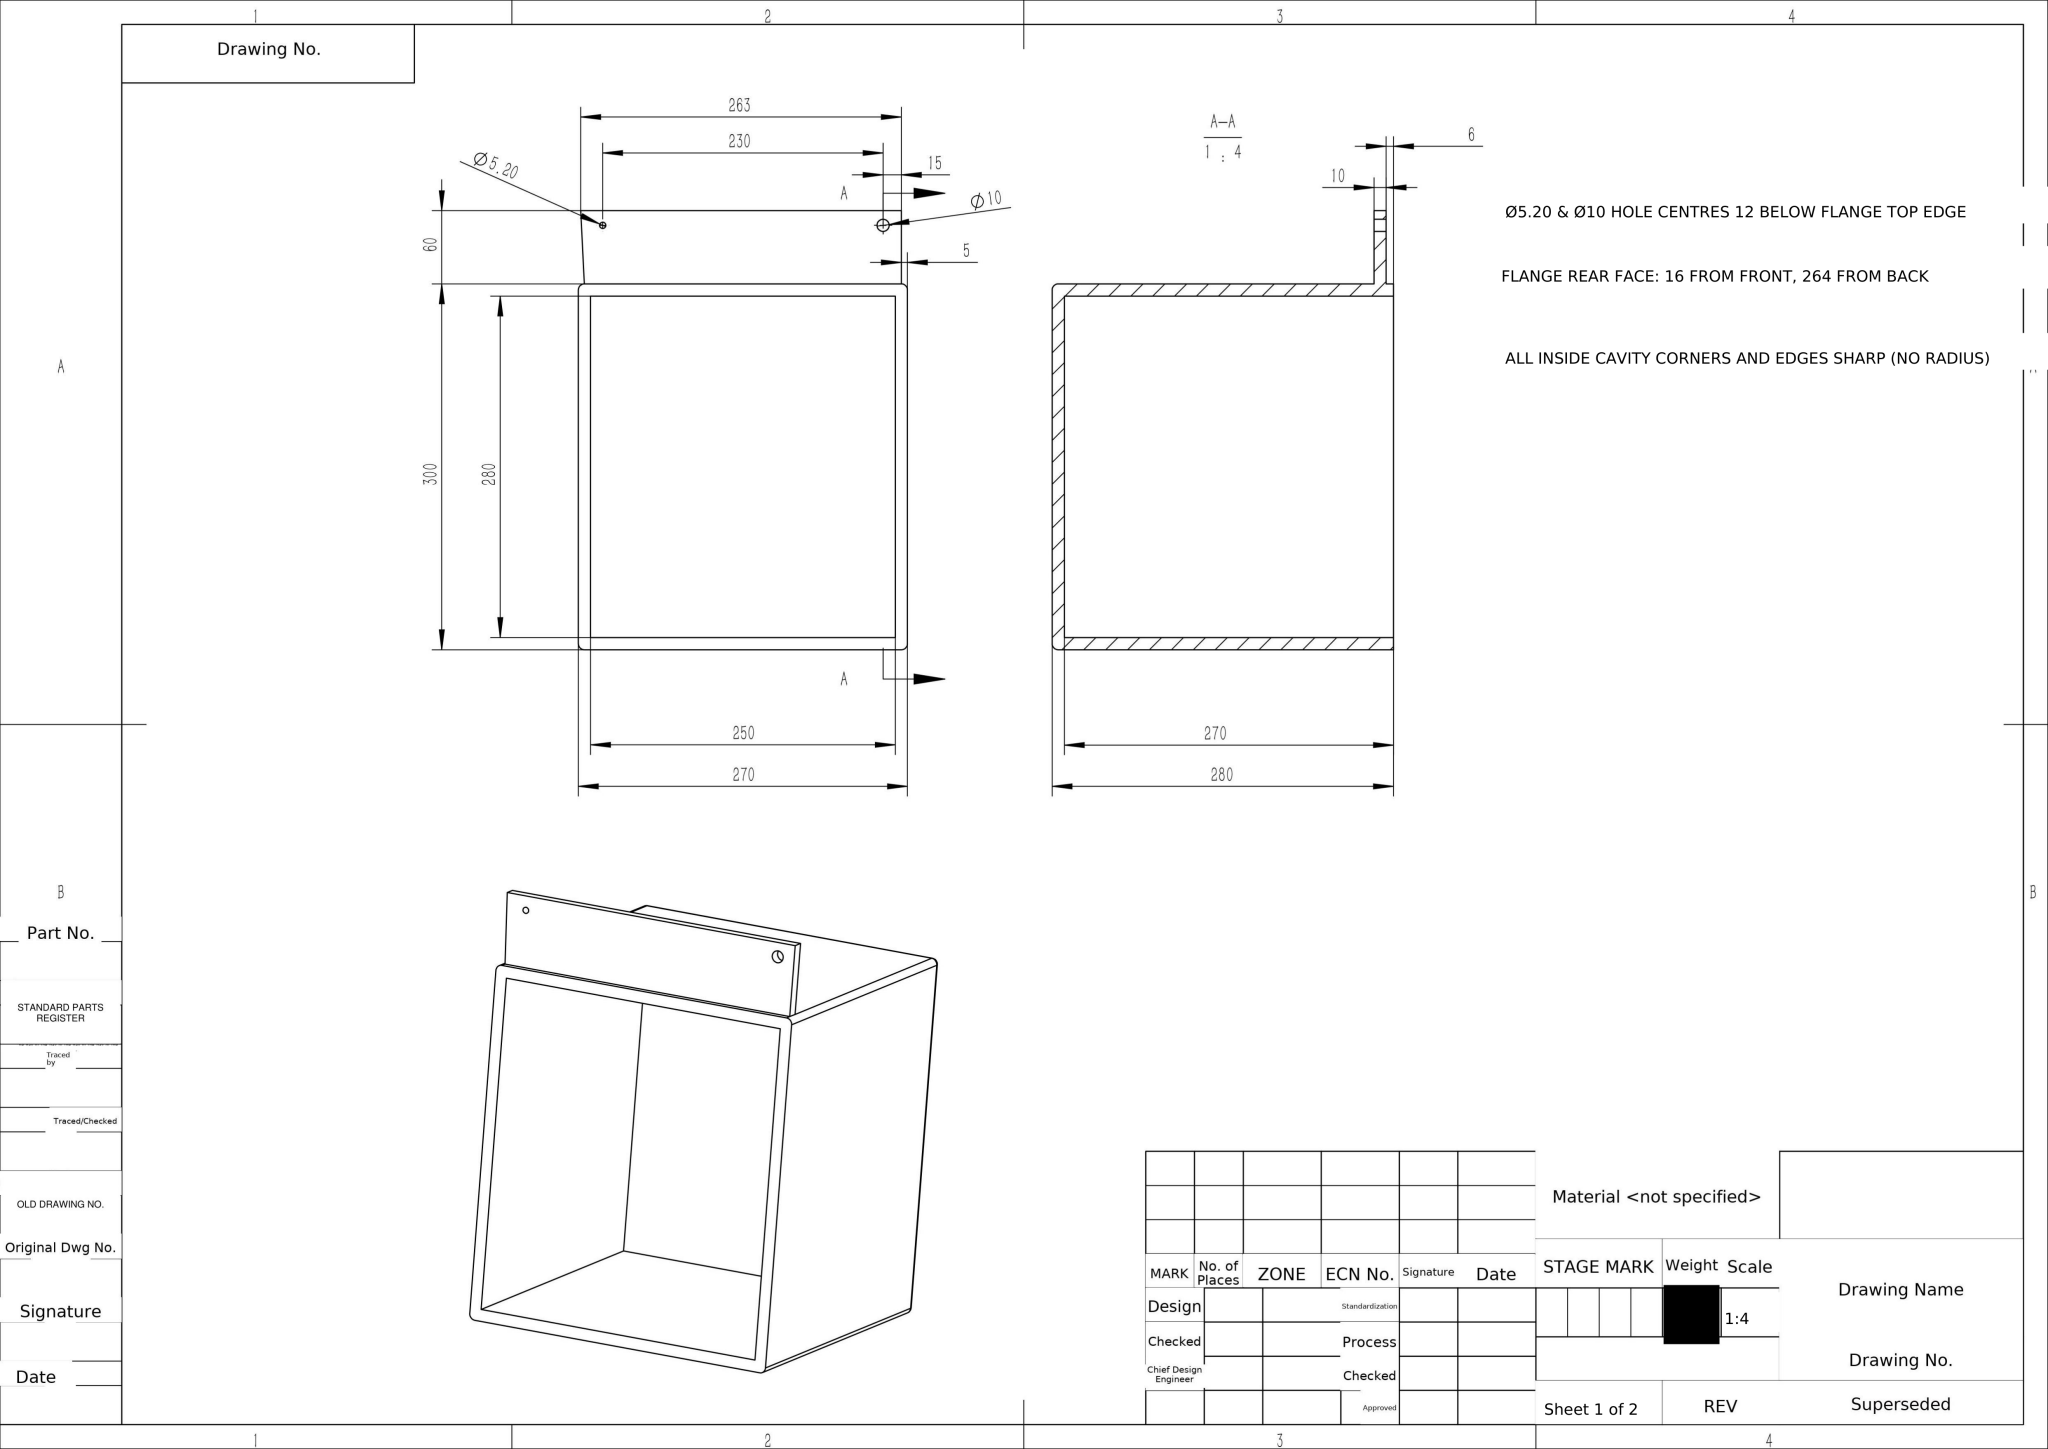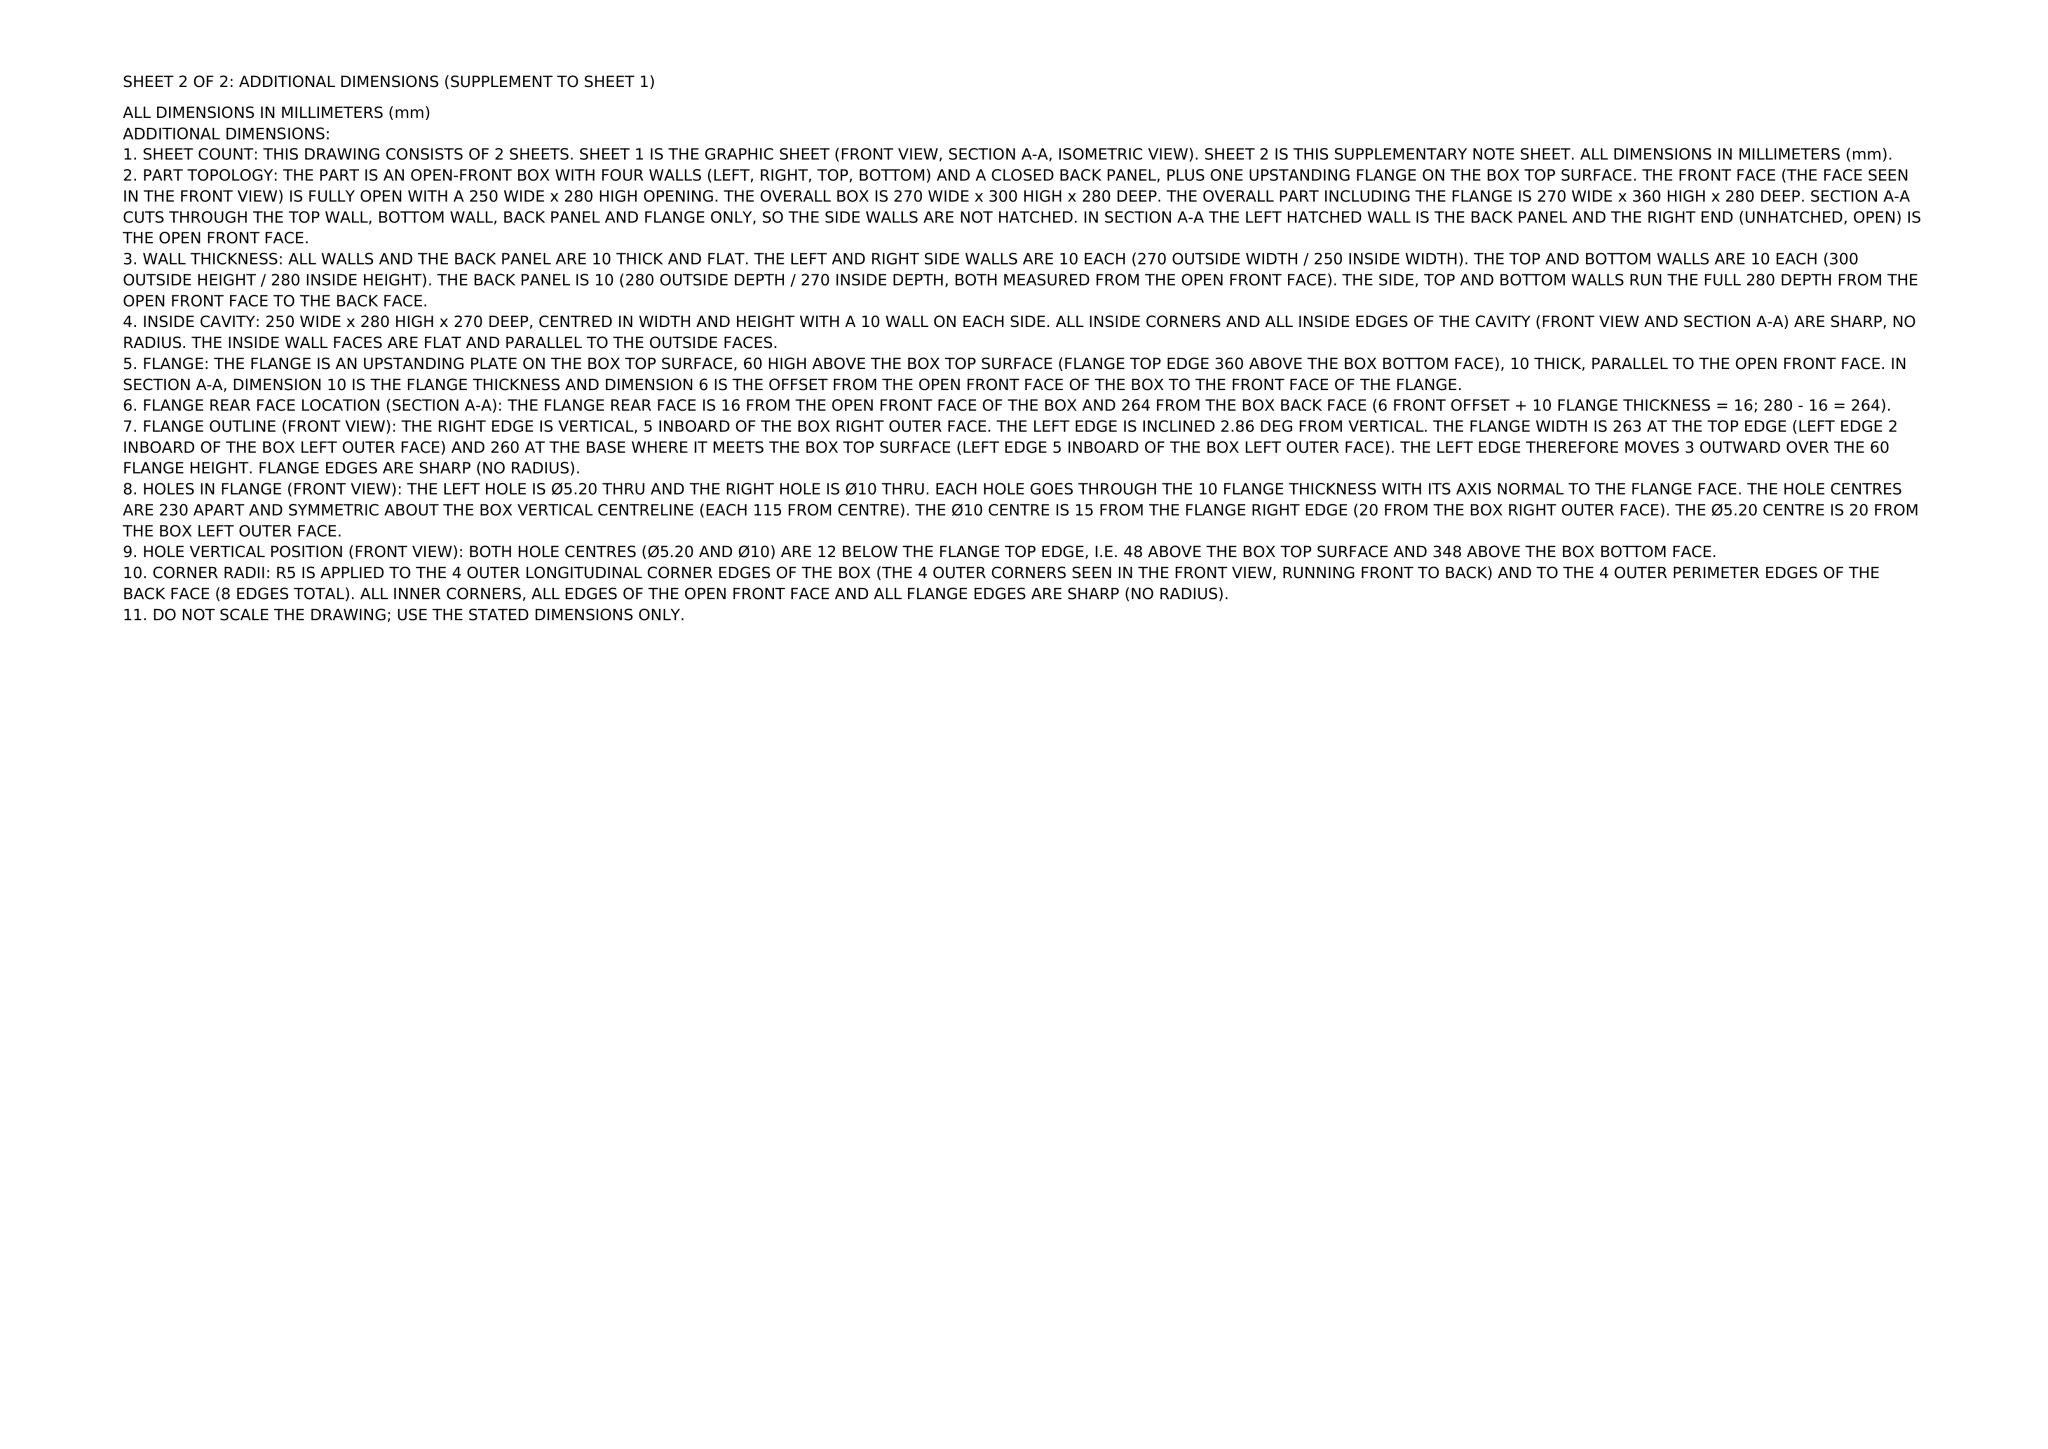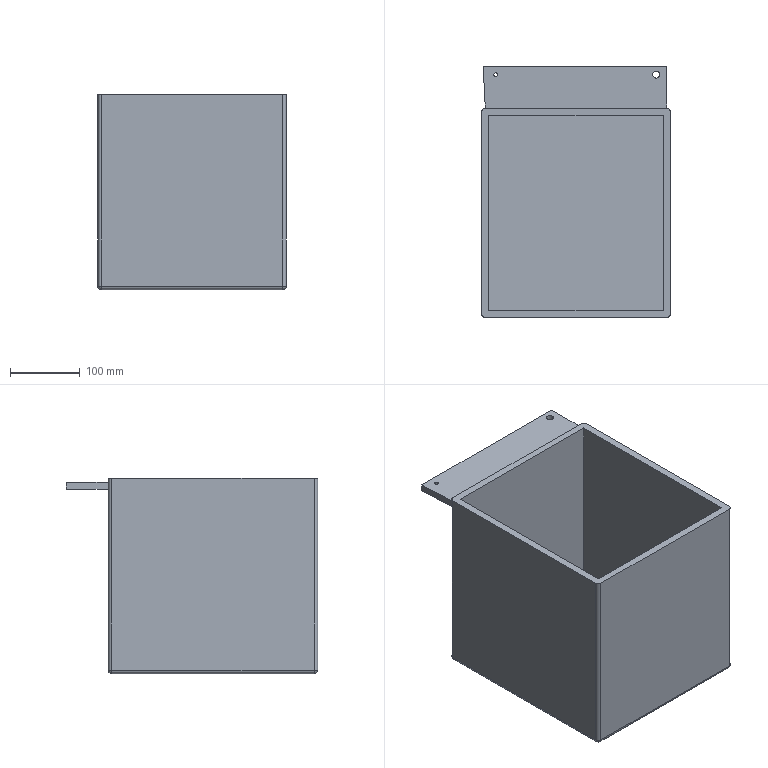Part | NX | mm | 1 solid | 33 faces | box 270 x 360 x 280 mm | volume 3923861 mm3 | plane 17 | cylinder 12 | sphere 4 | commonest cylinder face diameters 10 x10 5.2 x2